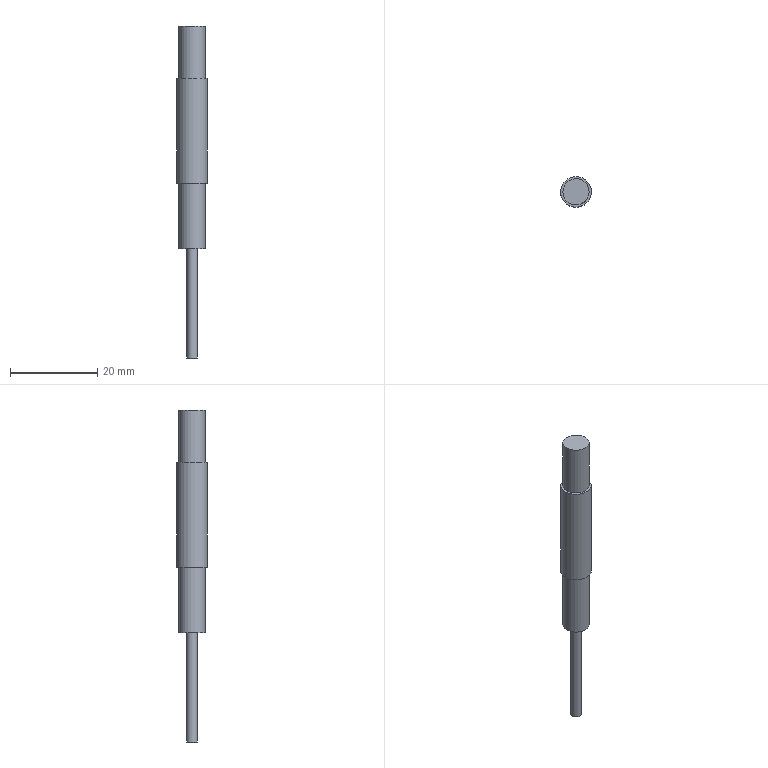Component | NX | DRIVEN_SHAFT | 1 solid | 9 faces | box 7 x 7 x 76 mm | volume 1810 mm3 | plane 5 | cylinder 4 | commonest cylinder face diameters 6 x2 7 x1 2.5 x1
STEP:
#1=CARTESIAN_POINT('',(0.,0.,0.));
#2=DIRECTION('',(0.,0.,1.));
#3=DIRECTION('',(1.,0.,0.));
#4=AXIS2_PLACEMENT_3D('',#1,#2,#3);
#5=CARTESIAN_POINT('',(8.702,0.6516,44.));
#6=VERTEX_POINT('',#5);
#7=CARTESIAN_POINT('',(5.266,-0.01624,44.));
#8=DIRECTION('',(0.,0.,1.));
#9=DIRECTION('',(0.9816,0.1908,0.));
#10=AXIS2_PLACEMENT_3D('',#7,#8,#9);
#11=CIRCLE('',#10,3.5);
#12=CARTESIAN_POINT('',(4.694,2.929,44.));
#13=DIRECTION('',(0.,0.,1.));
#14=DIRECTION('',(0.9816,0.1908,0.));
#15=AXIS2_PLACEMENT_3D('',#12,#13,#14);
#16=PLANE('',#15);
#17=CARTESIAN_POINT('',(-0.,-3.));
#18=DIRECTION('',(1.,0.));
#19=AXIS2_PLACEMENT_2D('',#17,#18);
#20=CIRCLE('',#19,3.5);
#21=(GEOMETRIC_REPRESENTATION_CONTEXT(2)PARAMETRIC_REPRESENTATION_CONTEXT()REPRESENTATION_CONTEXT('',''));
#22=DEFINITIONAL_REPRESENTATION('',(#20),#21);
#23=PCURVE('',#16,#22);
#24=CARTESIAN_POINT('',(5.266,-0.01624,56.));
#25=DIRECTION('',(0.,0.,1.));
#26=DIRECTION('',(0.9816,0.1908,0.));
#27=AXIS2_PLACEMENT_3D('',#24,#25,#26);
#28=CYLINDRICAL_SURFACE('',#27,3.5);
#29=CARTESIAN_POINT('',(0.,-12.));
#30=DIRECTION('',(1.,0.));
#31=VECTOR('',#30,1.);
#32=LINE('',#29,#31);
#33=(GEOMETRIC_REPRESENTATION_CONTEXT(2)PARAMETRIC_REPRESENTATION_CONTEXT()REPRESENTATION_CONTEXT('',''));
#34=DEFINITIONAL_REPRESENTATION('',(#32),#33);
#35=PCURVE('',#28,#34);
#36=SURFACE_CURVE('',#11,(#23,#35),.PCURVE_S1.);
#37=EDGE_CURVE('',#6,#6,#36,.T.);
#38=ORIENTED_EDGE('',*,*,#37,.T.);
#39=EDGE_LOOP('',(#38));
#40=FACE_BOUND('',#39,.T.);
#41=CARTESIAN_POINT('',(8.211,0.5562,44.));
#42=VERTEX_POINT('',#41);
#43=CARTESIAN_POINT('',(5.266,-0.01624,44.));
#44=DIRECTION('',(0.,0.,1.));
#45=DIRECTION('',(0.9816,0.1908,0.));
#46=AXIS2_PLACEMENT_3D('',#43,#44,#45);
#47=CIRCLE('',#46,3.);
#48=CARTESIAN_POINT('',(-0.,-3.));
#49=DIRECTION('',(1.,0.));
#50=AXIS2_PLACEMENT_2D('',#48,#49);
#51=CIRCLE('',#50,3.);
#52=(GEOMETRIC_REPRESENTATION_CONTEXT(2)PARAMETRIC_REPRESENTATION_CONTEXT()REPRESENTATION_CONTEXT('',''));
#53=DEFINITIONAL_REPRESENTATION('',(#51),#52);
#54=PCURVE('',#16,#53);
#55=CARTESIAN_POINT('',(5.266,-0.01624,56.));
#56=DIRECTION('',(0.,0.,1.));
#57=DIRECTION('',(0.9816,0.1908,0.));
#58=AXIS2_PLACEMENT_3D('',#55,#56,#57);
#59=CYLINDRICAL_SURFACE('',#58,3.);
#60=CARTESIAN_POINT('',(0.,-12.));
#61=DIRECTION('',(1.,0.));
#62=VECTOR('',#61,1.);
#63=LINE('',#60,#62);
#64=(GEOMETRIC_REPRESENTATION_CONTEXT(2)PARAMETRIC_REPRESENTATION_CONTEXT()REPRESENTATION_CONTEXT('',''));
#65=DEFINITIONAL_REPRESENTATION('',(#63),#64);
#66=PCURVE('',#59,#65);
#67=SURFACE_CURVE('',#47,(#54,#66),.PCURVE_S1.);
#68=EDGE_CURVE('',#42,#42,#67,.T.);
#69=ORIENTED_EDGE('',*,*,#68,.F.);
#70=EDGE_LOOP('',(#69));
#71=FACE_BOUND('',#70,.T.);
#72=ADVANCED_FACE('',(#40,#71),#16,.T.);
#73=CARTESIAN_POINT('',(8.702,0.6516,20.));
#74=VERTEX_POINT('',#73);
#75=CARTESIAN_POINT('',(5.266,-0.01624,20.));
#76=DIRECTION('',(0.,0.,1.));
#77=DIRECTION('',(0.9816,0.1908,0.));
#78=AXIS2_PLACEMENT_3D('',#75,#76,#77);
#79=CIRCLE('',#78,3.5);
#80=CARTESIAN_POINT('',(0.,-36.));
#81=DIRECTION('',(1.,0.));
#82=VECTOR('',#81,1.);
#83=LINE('',#80,#82);
#84=(GEOMETRIC_REPRESENTATION_CONTEXT(2)PARAMETRIC_REPRESENTATION_CONTEXT()REPRESENTATION_CONTEXT('',''));
#85=DEFINITIONAL_REPRESENTATION('',(#83),#84);
#86=PCURVE('',#28,#85);
#87=CARTESIAN_POINT('',(4.598,3.419,20.));
#88=DIRECTION('',(0.,0.,-1.));
#89=DIRECTION('',(-0.9816,-0.1908,0.));
#90=AXIS2_PLACEMENT_3D('',#87,#88,#89);
#91=PLANE('',#90);
#92=CARTESIAN_POINT('',(-3.5,-3.5));
#93=CARTESIAN_POINT('',(-3.5,2.562));
#94=CARTESIAN_POINT('',(1.75,-0.4689));
#95=CARTESIAN_POINT('',(7.,-3.5));
#96=CARTESIAN_POINT('',(1.75,-6.531));
#97=CARTESIAN_POINT('',(-3.5,-9.562));
#98=CARTESIAN_POINT('',(-3.5,-3.5));
#99=(BOUNDED_CURVE()B_SPLINE_CURVE(2,(#92,#93,#94,#95,#96,#97,#98),.UNSPECIFIED.,.T.,.F.)B_SPLINE_CURVE_WITH_KNOTS((1,2,2,2,2,1),(-2.094,0.,2.094,4.189,6.283,8.378),.UNSPECIFIED.)CURVE()GEOMETRIC_REPRESENTATION_ITEM()RATIONAL_B_SPLINE_CURVE((1.,0.5,1.,0.5,1.,0.5,1.))REPRESENTATION_ITEM(''));
#100=(GEOMETRIC_REPRESENTATION_CONTEXT(2)PARAMETRIC_REPRESENTATION_CONTEXT()REPRESENTATION_CONTEXT('',''));
#101=DEFINITIONAL_REPRESENTATION('',(#99),#100);
#102=PCURVE('',#91,#101);
#103=SURFACE_CURVE('',#79,(#86,#102),.PCURVE_S1.);
#104=EDGE_CURVE('',#74,#74,#103,.T.);
#105=ORIENTED_EDGE('',*,*,#104,.T.);
#106=CARTESIAN_POINT('',(8.702,0.6516,20.));
#107=CARTESIAN_POINT('',(8.702,0.6516,44.));
#108=B_SPLINE_CURVE_WITH_KNOTS('',1,(#106,#107),.UNSPECIFIED.,.F.,.F.,(2,2),(-36.,-12.),.PIECEWISE_BEZIER_KNOTS.);
#109=CARTESIAN_POINT('',(6.283,0.));
#110=DIRECTION('',(0.,1.));
#111=VECTOR('',#110,1.);
#112=LINE('',#109,#111);
#113=(GEOMETRIC_REPRESENTATION_CONTEXT(2)PARAMETRIC_REPRESENTATION_CONTEXT()REPRESENTATION_CONTEXT('',''));
#114=DEFINITIONAL_REPRESENTATION('',(#112),#113);
#115=PCURVE('',#28,#114);
#116=CARTESIAN_POINT('',(0.,0.));
#117=DIRECTION('',(0.,1.));
#118=VECTOR('',#117,1.);
#119=LINE('',#116,#118);
#120=(GEOMETRIC_REPRESENTATION_CONTEXT(2)PARAMETRIC_REPRESENTATION_CONTEXT()REPRESENTATION_CONTEXT('',''));
#121=DEFINITIONAL_REPRESENTATION('',(#119),#120);
#122=PCURVE('',#28,#121);
#123=SEAM_CURVE('',#108,(#115,#122),.PCURVE_S1.);
#124=EDGE_CURVE('',#74,#6,#123,.T.);
#125=ORIENTED_EDGE('',*,*,#124,.T.);
#126=ORIENTED_EDGE('',*,*,#37,.F.);
#127=ORIENTED_EDGE('',*,*,#124,.F.);
#128=EDGE_LOOP('',(#105,#125,#126,#127));
#129=FACE_BOUND('',#128,.T.);
#130=ADVANCED_FACE('',(#129),#28,.T.);
#131=CARTESIAN_POINT('',(8.211,0.5562,20.));
#132=VERTEX_POINT('',#131);
#133=CARTESIAN_POINT('',(5.266,-0.01624,20.));
#134=DIRECTION('',(0.,0.,1.));
#135=DIRECTION('',(0.9816,0.1908,0.));
#136=AXIS2_PLACEMENT_3D('',#133,#134,#135);
#137=CIRCLE('',#136,3.);
#138=CARTESIAN_POINT('',(-3.,-3.5));
#139=CARTESIAN_POINT('',(-3.,1.696));
#140=CARTESIAN_POINT('',(1.5,-0.9019));
#141=CARTESIAN_POINT('',(6.,-3.5));
#142=CARTESIAN_POINT('',(1.5,-6.098));
#143=CARTESIAN_POINT('',(-3.,-8.696));
#144=CARTESIAN_POINT('',(-3.,-3.5));
#145=(BOUNDED_CURVE()B_SPLINE_CURVE(2,(#138,#139,#140,#141,#142,#143,#144),.UNSPECIFIED.,.T.,.F.)B_SPLINE_CURVE_WITH_KNOTS((1,2,2,2,2,1),(-2.094,0.,2.094,4.189,6.283,8.378),.UNSPECIFIED.)CURVE()GEOMETRIC_REPRESENTATION_ITEM()RATIONAL_B_SPLINE_CURVE((1.,0.5,1.,0.5,1.,0.5,1.))REPRESENTATION_ITEM(''));
#146=(GEOMETRIC_REPRESENTATION_CONTEXT(2)PARAMETRIC_REPRESENTATION_CONTEXT()REPRESENTATION_CONTEXT('',''));
#147=DEFINITIONAL_REPRESENTATION('',(#145),#146);
#148=PCURVE('',#91,#147);
#149=CARTESIAN_POINT('',(5.266,-0.01624,56.));
#150=DIRECTION('',(0.,0.,1.));
#151=DIRECTION('',(0.9816,0.1908,0.));
#152=AXIS2_PLACEMENT_3D('',#149,#150,#151);
#153=CYLINDRICAL_SURFACE('',#152,3.);
#154=CARTESIAN_POINT('',(0.,-36.));
#155=DIRECTION('',(1.,0.));
#156=VECTOR('',#155,1.);
#157=LINE('',#154,#156);
#158=(GEOMETRIC_REPRESENTATION_CONTEXT(2)PARAMETRIC_REPRESENTATION_CONTEXT()REPRESENTATION_CONTEXT('',''));
#159=DEFINITIONAL_REPRESENTATION('',(#157),#158);
#160=PCURVE('',#153,#159);
#161=SURFACE_CURVE('',#137,(#148,#160),.PCURVE_S1.);
#162=EDGE_CURVE('',#132,#132,#161,.T.);
#163=ORIENTED_EDGE('',*,*,#162,.T.);
#164=EDGE_LOOP('',(#163));
#165=FACE_BOUND('',#164,.T.);
#166=ORIENTED_EDGE('',*,*,#104,.F.);
#167=EDGE_LOOP('',(#166));
#168=FACE_BOUND('',#167,.T.);
#169=ADVANCED_FACE('',(#165,#168),#91,.T.);
#170=ORIENTED_EDGE('',*,*,#162,.F.);
#171=CARTESIAN_POINT('',(8.211,0.5562,5.));
#172=VERTEX_POINT('',#171);
#173=CARTESIAN_POINT('',(8.211,0.5562,5.));
#174=CARTESIAN_POINT('',(8.211,0.5562,20.));
#175=B_SPLINE_CURVE_WITH_KNOTS('',1,(#173,#174),.UNSPECIFIED.,.F.,.F.,(2,2),(-51.,-36.),.PIECEWISE_BEZIER_KNOTS.);
#176=CARTESIAN_POINT('',(0.,0.));
#177=DIRECTION('',(0.,1.));
#178=VECTOR('',#177,1.);
#179=LINE('',#176,#178);
#180=(GEOMETRIC_REPRESENTATION_CONTEXT(2)PARAMETRIC_REPRESENTATION_CONTEXT()REPRESENTATION_CONTEXT('',''));
#181=DEFINITIONAL_REPRESENTATION('',(#179),#180);
#182=PCURVE('',#153,#181);
#183=CARTESIAN_POINT('',(6.283,0.));
#184=DIRECTION('',(0.,1.));
#185=VECTOR('',#184,1.);
#186=LINE('',#183,#185);
#187=(GEOMETRIC_REPRESENTATION_CONTEXT(2)PARAMETRIC_REPRESENTATION_CONTEXT()REPRESENTATION_CONTEXT('',''));
#188=DEFINITIONAL_REPRESENTATION('',(#186),#187);
#189=PCURVE('',#153,#188);
#190=SEAM_CURVE('',#175,(#182,#189),.PCURVE_S1.);
#191=EDGE_CURVE('',#172,#132,#190,.T.);
#192=ORIENTED_EDGE('',*,*,#191,.F.);
#193=CARTESIAN_POINT('',(5.266,-0.01624,5.));
#194=DIRECTION('',(0.,0.,-1.));
#195=DIRECTION('',(0.9816,0.1908,0.));
#196=AXIS2_PLACEMENT_3D('',#193,#194,#195);
#197=CIRCLE('',#196,3.);
#198=CARTESIAN_POINT('',(6.283,-51.));
#199=DIRECTION('',(-1.,0.));
#200=VECTOR('',#199,1.);
#201=LINE('',#198,#200);
#202=(GEOMETRIC_REPRESENTATION_CONTEXT(2)PARAMETRIC_REPRESENTATION_CONTEXT()REPRESENTATION_CONTEXT('',''));
#203=DEFINITIONAL_REPRESENTATION('',(#201),#202);
#204=PCURVE('',#153,#203);
#205=CARTESIAN_POINT('',(5.266,-0.01624,5.));
#206=DIRECTION('',(0.,0.,-1.));
#207=DIRECTION('',(-0.9816,-0.1908,0.));
#208=AXIS2_PLACEMENT_3D('',#205,#206,#207);
#209=PLANE('',#208);
#210=CARTESIAN_POINT('',(0.,0.));
#211=DIRECTION('',(-1.,0.));
#212=AXIS2_PLACEMENT_2D('',#210,#211);
#213=CIRCLE('',#212,3.);
#214=(GEOMETRIC_REPRESENTATION_CONTEXT(2)PARAMETRIC_REPRESENTATION_CONTEXT()REPRESENTATION_CONTEXT('',''));
#215=DEFINITIONAL_REPRESENTATION('',(#213),#214);
#216=PCURVE('',#209,#215);
#217=SURFACE_CURVE('',#197,(#204,#216),.PCURVE_S1.);
#218=EDGE_CURVE('',#172,#172,#217,.T.);
#219=ORIENTED_EDGE('',*,*,#218,.F.);
#220=ORIENTED_EDGE('',*,*,#191,.T.);
#221=EDGE_LOOP('',(#170,#192,#219,#220));
#222=FACE_BOUND('',#221,.T.);
#223=ADVANCED_FACE('',(#222),#153,.T.);
#224=CARTESIAN_POINT('',(8.211,0.5562,56.));
#225=VERTEX_POINT('',#224);
#226=CARTESIAN_POINT('',(5.266,-0.01624,56.));
#227=DIRECTION('',(0.,0.,1.));
#228=DIRECTION('',(0.9816,0.1908,0.));
#229=AXIS2_PLACEMENT_3D('',#226,#227,#228);
#230=CIRCLE('',#229,3.);
#231=CARTESIAN_POINT('',(5.266,-0.01624,56.));
#232=DIRECTION('',(0.,0.,1.));
#233=DIRECTION('',(0.9816,0.1908,0.));
#234=AXIS2_PLACEMENT_3D('',#231,#232,#233);
#235=PLANE('',#234);
#236=CARTESIAN_POINT('',(0.,0.));
#237=DIRECTION('',(1.,0.));
#238=AXIS2_PLACEMENT_2D('',#236,#237);
#239=CIRCLE('',#238,3.);
#240=(GEOMETRIC_REPRESENTATION_CONTEXT(2)PARAMETRIC_REPRESENTATION_CONTEXT()REPRESENTATION_CONTEXT('',''));
#241=DEFINITIONAL_REPRESENTATION('',(#239),#240);
#242=PCURVE('',#235,#241);
#243=CARTESIAN_POINT('',(0.,0.));
#244=DIRECTION('',(1.,0.));
#245=VECTOR('',#244,1.);
#246=LINE('',#243,#245);
#247=(GEOMETRIC_REPRESENTATION_CONTEXT(2)PARAMETRIC_REPRESENTATION_CONTEXT()REPRESENTATION_CONTEXT('',''));
#248=DEFINITIONAL_REPRESENTATION('',(#246),#247);
#249=PCURVE('',#59,#248);
#250=SURFACE_CURVE('',#230,(#242,#249),.PCURVE_S1.);
#251=EDGE_CURVE('',#225,#225,#250,.T.);
#252=ORIENTED_EDGE('',*,*,#251,.T.);
#253=EDGE_LOOP('',(#252));
#254=FACE_BOUND('',#253,.T.);
#255=ADVANCED_FACE('',(#254),#235,.T.);
#256=ORIENTED_EDGE('',*,*,#68,.T.);
#257=CARTESIAN_POINT('',(8.211,0.5562,44.));
#258=CARTESIAN_POINT('',(8.211,0.5562,56.));
#259=B_SPLINE_CURVE_WITH_KNOTS('',1,(#257,#258),.UNSPECIFIED.,.F.,.F.,(2,2),(-12.,0.),.PIECEWISE_BEZIER_KNOTS.);
#260=CARTESIAN_POINT('',(6.283,0.));
#261=DIRECTION('',(0.,1.));
#262=VECTOR('',#261,1.);
#263=LINE('',#260,#262);
#264=(GEOMETRIC_REPRESENTATION_CONTEXT(2)PARAMETRIC_REPRESENTATION_CONTEXT()REPRESENTATION_CONTEXT('',''));
#265=DEFINITIONAL_REPRESENTATION('',(#263),#264);
#266=PCURVE('',#59,#265);
#267=CARTESIAN_POINT('',(0.,0.));
#268=DIRECTION('',(0.,1.));
#269=VECTOR('',#268,1.);
#270=LINE('',#267,#269);
#271=(GEOMETRIC_REPRESENTATION_CONTEXT(2)PARAMETRIC_REPRESENTATION_CONTEXT()REPRESENTATION_CONTEXT('',''));
#272=DEFINITIONAL_REPRESENTATION('',(#270),#271);
#273=PCURVE('',#59,#272);
#274=SEAM_CURVE('',#259,(#266,#273),.PCURVE_S1.);
#275=EDGE_CURVE('',#42,#225,#274,.T.);
#276=ORIENTED_EDGE('',*,*,#275,.T.);
#277=ORIENTED_EDGE('',*,*,#251,.F.);
#278=ORIENTED_EDGE('',*,*,#275,.F.);
#279=EDGE_LOOP('',(#256,#276,#277,#278));
#280=FACE_BOUND('',#279,.T.);
#281=ADVANCED_FACE('',(#280),#59,.T.);
#282=CARTESIAN_POINT('',(4.039,-0.2548,5.));
#283=VERTEX_POINT('',#282);
#284=CARTESIAN_POINT('',(6.493,0.2223,5.));
#285=VERTEX_POINT('',#284);
#286=CARTESIAN_POINT('',(5.266,-0.01624,5.));
#287=DIRECTION('',(0.,0.,1.));
#288=DIRECTION('',(-0.9816,-0.1908,0.));
#289=AXIS2_PLACEMENT_3D('',#286,#287,#288);
#290=CIRCLE('',#289,1.25);
#291=CARTESIAN_POINT('',(1.25,0.));
#292=CARTESIAN_POINT('',(1.25,-2.165));
#293=CARTESIAN_POINT('',(-0.625,-1.083));
#294=CARTESIAN_POINT('',(-2.5,-0.));
#295=CARTESIAN_POINT('',(-0.625,1.083));
#296=CARTESIAN_POINT('',(1.25,2.165));
#297=CARTESIAN_POINT('',(1.25,0.));
#298=(BOUNDED_CURVE()B_SPLINE_CURVE(2,(#291,#292,#293,#294,#295,#296,#297),.UNSPECIFIED.,.T.,.F.)B_SPLINE_CURVE_WITH_KNOTS((1,2,2,2,2,1),(-2.094,0.,2.094,4.189,6.283,8.378),.UNSPECIFIED.)CURVE()GEOMETRIC_REPRESENTATION_ITEM()RATIONAL_B_SPLINE_CURVE((1.,0.5,1.,0.5,1.,0.5,1.))REPRESENTATION_ITEM(''));
#299=(GEOMETRIC_REPRESENTATION_CONTEXT(2)PARAMETRIC_REPRESENTATION_CONTEXT()REPRESENTATION_CONTEXT('',''));
#300=DEFINITIONAL_REPRESENTATION('',(#298),#299);
#301=PCURVE('',#209,#300);
#302=CARTESIAN_POINT('',(5.266,-0.01624,56.));
#303=DIRECTION('',(0.,0.,1.));
#304=DIRECTION('',(0.9816,0.1908,0.));
#305=AXIS2_PLACEMENT_3D('',#302,#303,#304);
#306=CYLINDRICAL_SURFACE('',#305,1.25);
#307=CARTESIAN_POINT('',(3.142,-51.));
#308=DIRECTION('',(1.,0.));
#309=VECTOR('',#308,1.);
#310=LINE('',#307,#309);
#311=(GEOMETRIC_REPRESENTATION_CONTEXT(2)PARAMETRIC_REPRESENTATION_CONTEXT()REPRESENTATION_CONTEXT('',''));
#312=DEFINITIONAL_REPRESENTATION('',(#310),#311);
#313=PCURVE('',#306,#312);
#314=SURFACE_CURVE('',#290,(#301,#313),.PCURVE_S1.);
#315=EDGE_CURVE('',#283,#285,#314,.T.);
#316=ORIENTED_EDGE('',*,*,#315,.T.);
#317=CARTESIAN_POINT('',(5.266,-0.01624,5.));
#318=DIRECTION('',(0.,0.,1.));
#319=DIRECTION('',(-0.9816,-0.1908,0.));
#320=AXIS2_PLACEMENT_3D('',#317,#318,#319);
#321=CIRCLE('',#320,1.25);
#322=CARTESIAN_POINT('',(1.25,0.));
#323=CARTESIAN_POINT('',(1.25,-2.165));
#324=CARTESIAN_POINT('',(-0.625,-1.083));
#325=CARTESIAN_POINT('',(-2.5,-0.));
#326=CARTESIAN_POINT('',(-0.625,1.083));
#327=CARTESIAN_POINT('',(1.25,2.165));
#328=CARTESIAN_POINT('',(1.25,0.));
#329=(BOUNDED_CURVE()B_SPLINE_CURVE(2,(#322,#323,#324,#325,#326,#327,#328),.UNSPECIFIED.,.T.,.F.)B_SPLINE_CURVE_WITH_KNOTS((1,2,2,2,2,1),(-2.094,0.,2.094,4.189,6.283,8.378),.UNSPECIFIED.)CURVE()GEOMETRIC_REPRESENTATION_ITEM()RATIONAL_B_SPLINE_CURVE((1.,0.5,1.,0.5,1.,0.5,1.))REPRESENTATION_ITEM(''));
#330=(GEOMETRIC_REPRESENTATION_CONTEXT(2)PARAMETRIC_REPRESENTATION_CONTEXT()REPRESENTATION_CONTEXT('',''));
#331=DEFINITIONAL_REPRESENTATION('',(#329),#330);
#332=PCURVE('',#209,#331);
#333=CARTESIAN_POINT('',(-3.142,-51.));
#334=DIRECTION('',(1.,0.));
#335=VECTOR('',#334,1.);
#336=LINE('',#333,#335);
#337=(GEOMETRIC_REPRESENTATION_CONTEXT(2)PARAMETRIC_REPRESENTATION_CONTEXT()REPRESENTATION_CONTEXT('',''));
#338=DEFINITIONAL_REPRESENTATION('',(#336),#337);
#339=PCURVE('',#306,#338);
#340=SURFACE_CURVE('',#321,(#332,#339),.PCURVE_S1.);
#341=EDGE_CURVE('',#285,#283,#340,.T.);
#342=ORIENTED_EDGE('',*,*,#341,.T.);
#343=EDGE_LOOP('',(#316,#342));
#344=FACE_BOUND('',#343,.T.);
#345=ORIENTED_EDGE('',*,*,#218,.T.);
#346=EDGE_LOOP('',(#345));
#347=FACE_BOUND('',#346,.T.);
#348=ADVANCED_FACE('',(#344,#347),#209,.T.);
#349=CARTESIAN_POINT('',(6.493,0.2223,-20.));
#350=VERTEX_POINT('',#349);
#351=CARTESIAN_POINT('',(5.266,-0.01624,-20.));
#352=DIRECTION('',(0.,0.,1.));
#353=DIRECTION('',(0.9816,0.1908,0.));
#354=AXIS2_PLACEMENT_3D('',#351,#352,#353);
#355=CIRCLE('',#354,1.25);
#356=CARTESIAN_POINT('',(5.028,1.211,-20.));
#357=DIRECTION('',(0.,0.,-1.));
#358=DIRECTION('',(-0.9816,-0.1908,0.));
#359=AXIS2_PLACEMENT_3D('',#356,#357,#358);
#360=PLANE('',#359);
#361=CARTESIAN_POINT('',(-1.25,-1.25));
#362=CARTESIAN_POINT('',(-1.25,0.9151));
#363=CARTESIAN_POINT('',(0.625,-0.1675));
#364=CARTESIAN_POINT('',(2.5,-1.25));
#365=CARTESIAN_POINT('',(0.625,-2.333));
#366=CARTESIAN_POINT('',(-1.25,-3.415));
#367=CARTESIAN_POINT('',(-1.25,-1.25));
#368=(BOUNDED_CURVE()B_SPLINE_CURVE(2,(#361,#362,#363,#364,#365,#366,#367),.UNSPECIFIED.,.T.,.F.)B_SPLINE_CURVE_WITH_KNOTS((1,2,2,2,2,1),(-2.094,0.,2.094,4.189,6.283,8.378),.UNSPECIFIED.)CURVE()GEOMETRIC_REPRESENTATION_ITEM()RATIONAL_B_SPLINE_CURVE((1.,0.5,1.,0.5,1.,0.5,1.))REPRESENTATION_ITEM(''));
#369=(GEOMETRIC_REPRESENTATION_CONTEXT(2)PARAMETRIC_REPRESENTATION_CONTEXT()REPRESENTATION_CONTEXT('',''));
#370=DEFINITIONAL_REPRESENTATION('',(#368),#369);
#371=PCURVE('',#360,#370);
#372=CARTESIAN_POINT('',(0.,-76.));
#373=DIRECTION('',(1.,0.));
#374=VECTOR('',#373,1.);
#375=LINE('',#372,#374);
#376=(GEOMETRIC_REPRESENTATION_CONTEXT(2)PARAMETRIC_REPRESENTATION_CONTEXT()REPRESENTATION_CONTEXT('',''));
#377=DEFINITIONAL_REPRESENTATION('',(#375),#376);
#378=PCURVE('',#306,#377);
#379=SURFACE_CURVE('',#355,(#371,#378),.PCURVE_S1.);
#380=EDGE_CURVE('',#350,#350,#379,.T.);
#381=ORIENTED_EDGE('',*,*,#380,.F.);
#382=EDGE_LOOP('',(#381));
#383=FACE_BOUND('',#382,.T.);
#384=ADVANCED_FACE('',(#383),#360,.T.);
#385=ORIENTED_EDGE('',*,*,#341,.F.);
#386=CARTESIAN_POINT('',(6.493,0.2223,-20.));
#387=CARTESIAN_POINT('',(6.493,0.2223,5.));
#388=B_SPLINE_CURVE_WITH_KNOTS('',1,(#386,#387),.UNSPECIFIED.,.F.,.F.,(2,2),(-76.,-51.),.PIECEWISE_BEZIER_KNOTS.);
#389=CARTESIAN_POINT('',(0.,0.));
#390=DIRECTION('',(0.,1.));
#391=VECTOR('',#390,1.);
#392=LINE('',#389,#391);
#393=(GEOMETRIC_REPRESENTATION_CONTEXT(2)PARAMETRIC_REPRESENTATION_CONTEXT()REPRESENTATION_CONTEXT('',''));
#394=DEFINITIONAL_REPRESENTATION('',(#392),#393);
#395=PCURVE('',#306,#394);
#396=CARTESIAN_POINT('',(6.283,0.));
#397=DIRECTION('',(0.,1.));
#398=VECTOR('',#397,1.);
#399=LINE('',#396,#398);
#400=(GEOMETRIC_REPRESENTATION_CONTEXT(2)PARAMETRIC_REPRESENTATION_CONTEXT()REPRESENTATION_CONTEXT('',''));
#401=DEFINITIONAL_REPRESENTATION('',(#399),#400);
#402=PCURVE('',#306,#401);
#403=SEAM_CURVE('',#388,(#395,#402),.PCURVE_S1.);
#404=EDGE_CURVE('',#350,#285,#403,.T.);
#405=ORIENTED_EDGE('',*,*,#404,.F.);
#406=ORIENTED_EDGE('',*,*,#380,.T.);
#407=ORIENTED_EDGE('',*,*,#404,.T.);
#408=ORIENTED_EDGE('',*,*,#315,.F.);
#409=EDGE_LOOP('',(#385,#405,#406,#407,#408));
#410=FACE_BOUND('',#409,.T.);
#411=ADVANCED_FACE('',(#410),#306,.T.);
#412=CLOSED_SHELL('',(#72,#130,#169,#223,#255,#281,#348,#384,#411));
#413=MANIFOLD_SOLID_BREP('',#412);
#414=(LENGTH_UNIT()NAMED_UNIT(*)SI_UNIT(.MILLI.,.METRE.));
#415=UNCERTAINTY_MEASURE_WITH_UNIT(LENGTH_MEASURE(0.000005),#414,'','');
#416=(NAMED_UNIT(*)PLANE_ANGLE_UNIT()SI_UNIT($,.RADIAN.));
#417=(NAMED_UNIT(*)SI_UNIT($,.STERADIAN.)SOLID_ANGLE_UNIT());
#418=(GEOMETRIC_REPRESENTATION_CONTEXT(3)GLOBAL_UNCERTAINTY_ASSIGNED_CONTEXT((#415))GLOBAL_UNIT_ASSIGNED_CONTEXT((#414,#416,#417))REPRESENTATION_CONTEXT('',''));
#419=ADVANCED_BREP_SHAPE_REPRESENTATION('',(#4,#413),#418);